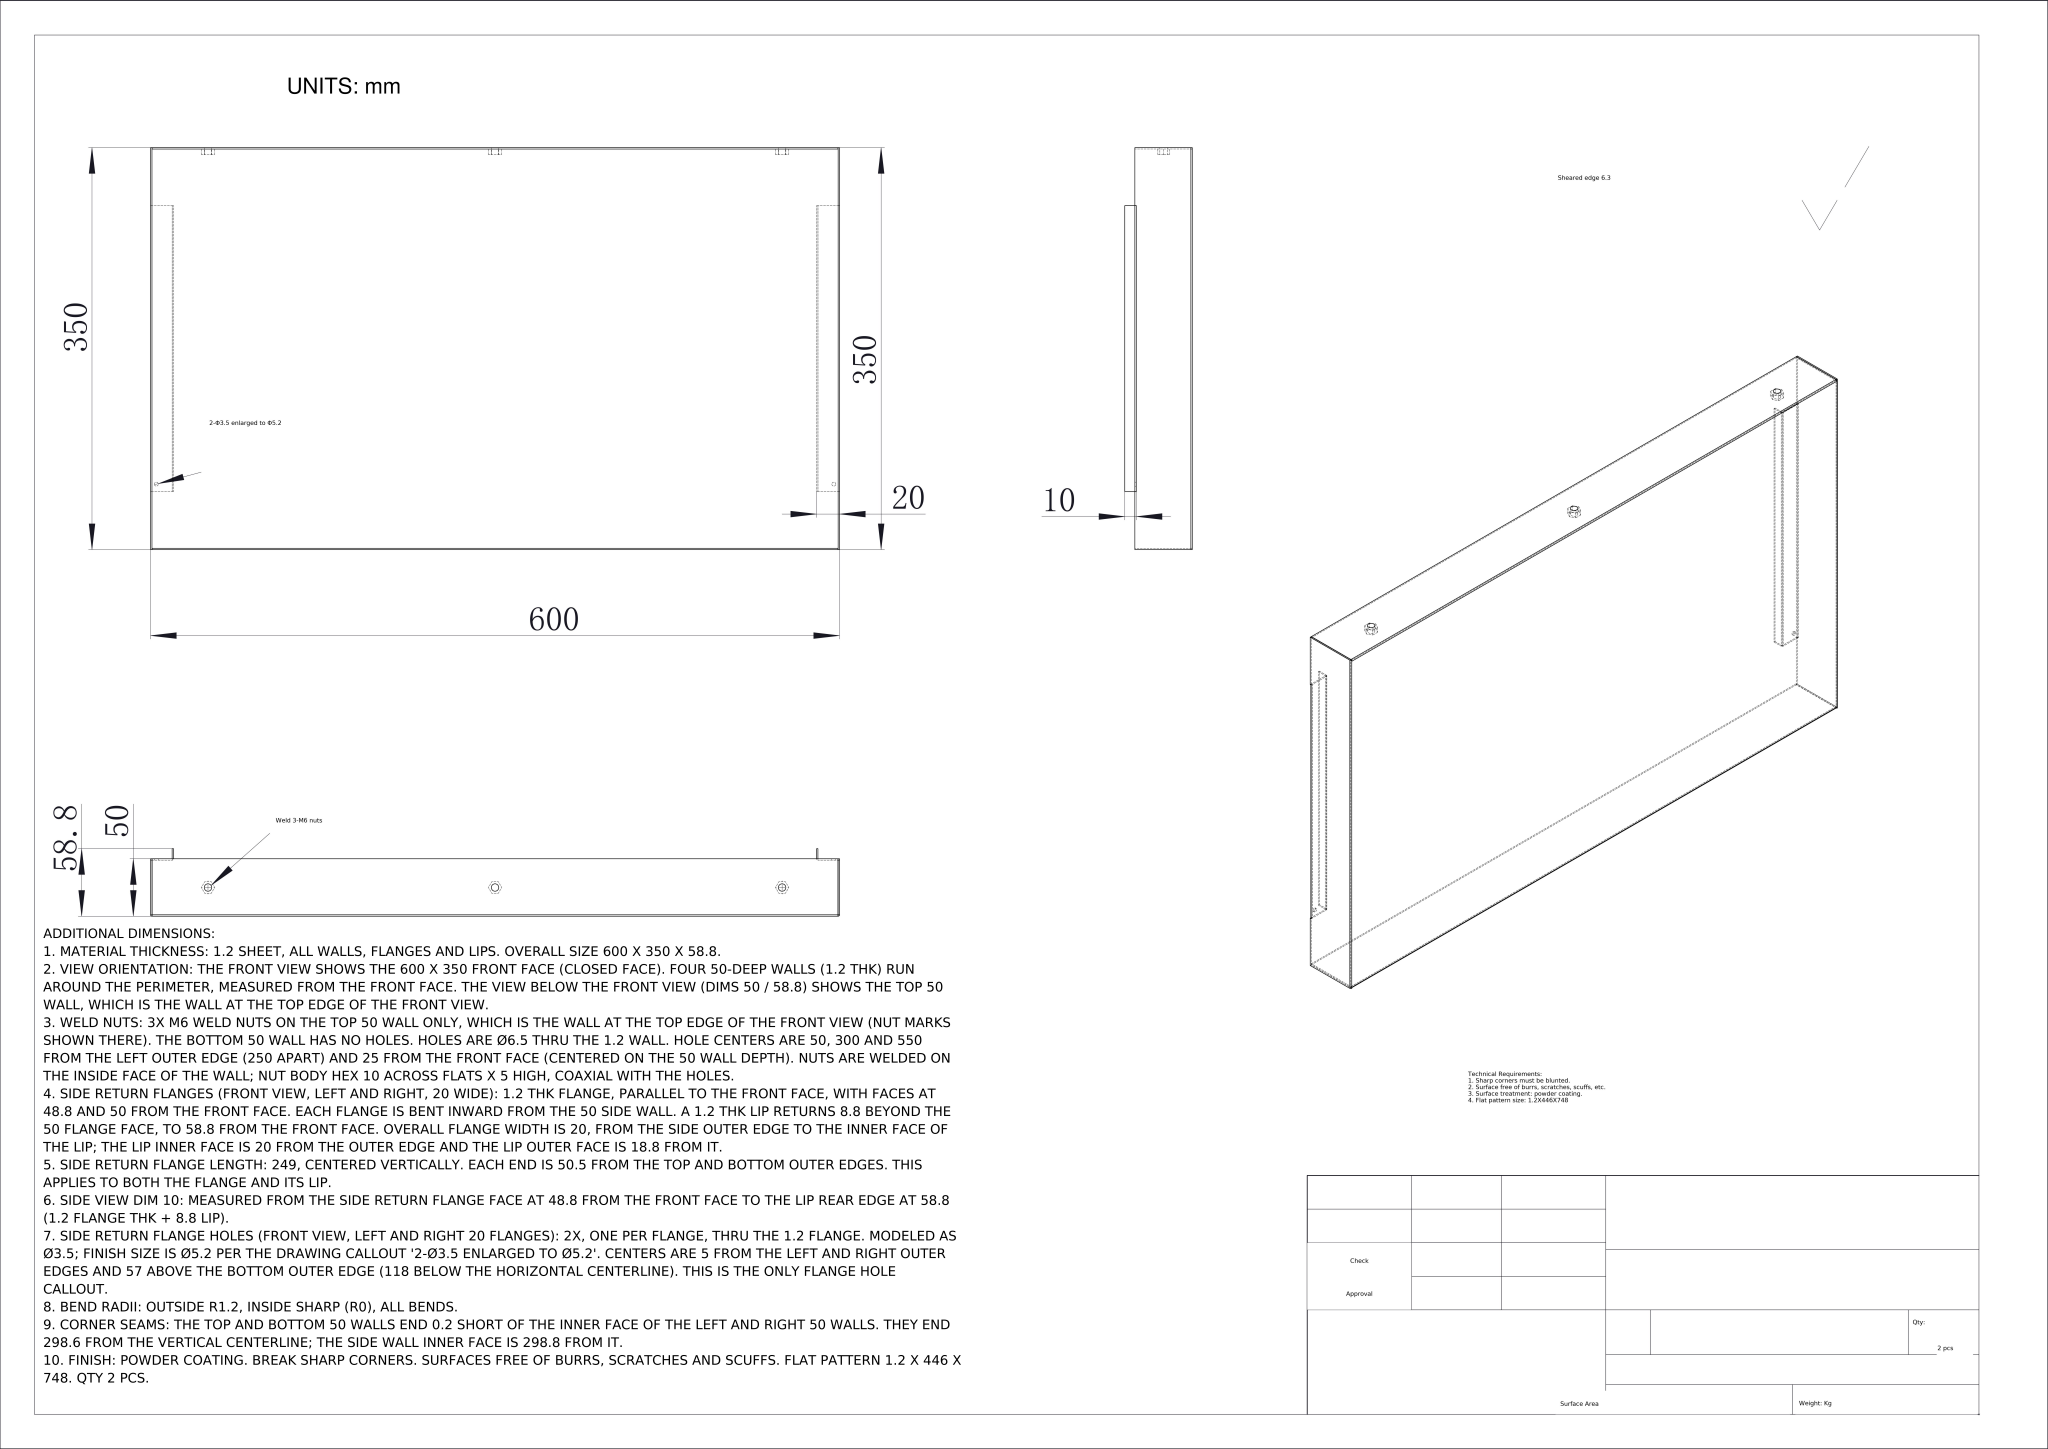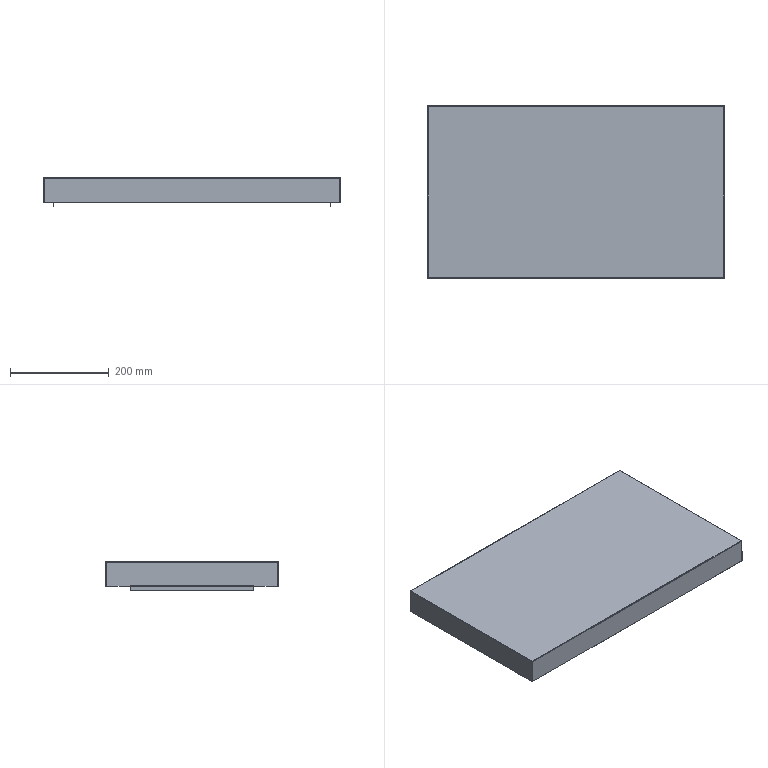Part | NX | mm | 1 solid | 135 faces | box 600 x 350 x 58.8 mm | volume 379193 mm3 | plane 99 | cylinder 36 | commonest cylinder face diameters 0.06 x10 2.402 x8 0.002 x8 6.5 x6 3.5 x4